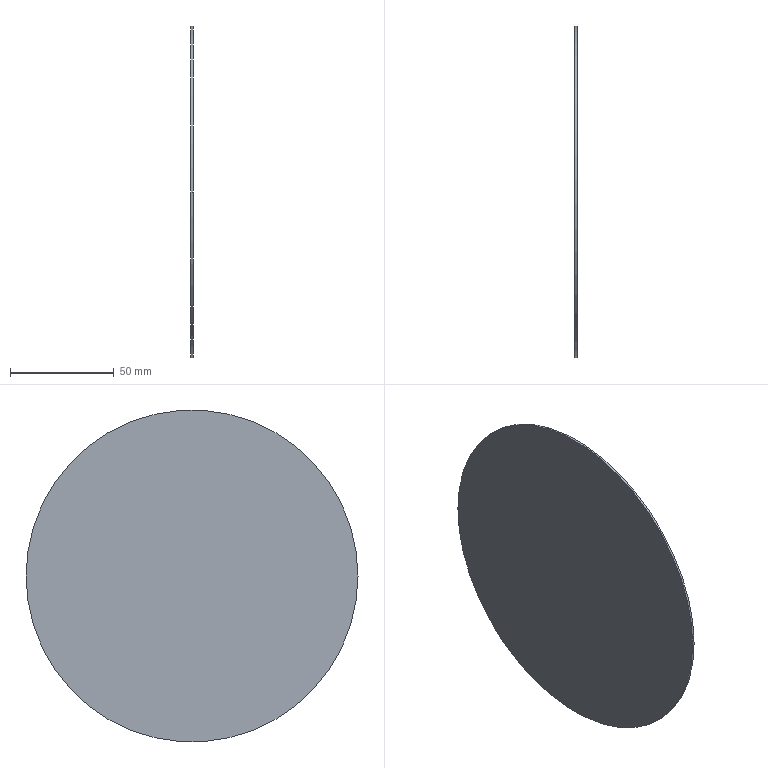Component | SolidWorks | Plate-1 | 1 solid | 4 faces | box 1 x 160 x 160 mm | volume 20106 mm3 | cylinder 2 | plane 2 | commonest cylinder face diameters 160 x2
build123d program:
from build123d import *

# Parameters (mm, degrees)
SKETCH1_W                          = 87.5
SKETCH1_H                          = 1
SKETCH2_R                          = 90
SKETCH2_R_2                        = 80
REPAIR_OD160TOFITCOUNTERBORE_DEPTH = 1.75


with BuildPart() as part:
    # Sketch1 → Revolve1 (revolve)
    with BuildSketch(Plane(origin=(0, 0, 0), x_dir=(1, 0, 0), z_dir=(0, 1, 0))):
        with Locations((43.75, 53.405)):
            Rectangle(SKETCH1_W, SKETCH1_H)
    revolve(axis=Axis((0, 0, -53.905), (0, 0, 1)))

    # Sketch2 → Repair_OD160ToFitCounterbore (cut, symmetric)
    with BuildSketch(Plane.XY.offset(-53.457)):
        Circle(SKETCH2_R)
        Circle(SKETCH2_R_2, mode=Mode.SUBTRACT)
    extrude(amount=REPAIR_OD160TOFITCOUNTERBORE_DEPTH, both=True, mode=Mode.SUBTRACT)


solid = part.part

# Placed as in the assembly
solid = solid.moved(Location((-722.896, 870.769, 1116.347), (0, 90, 0)))